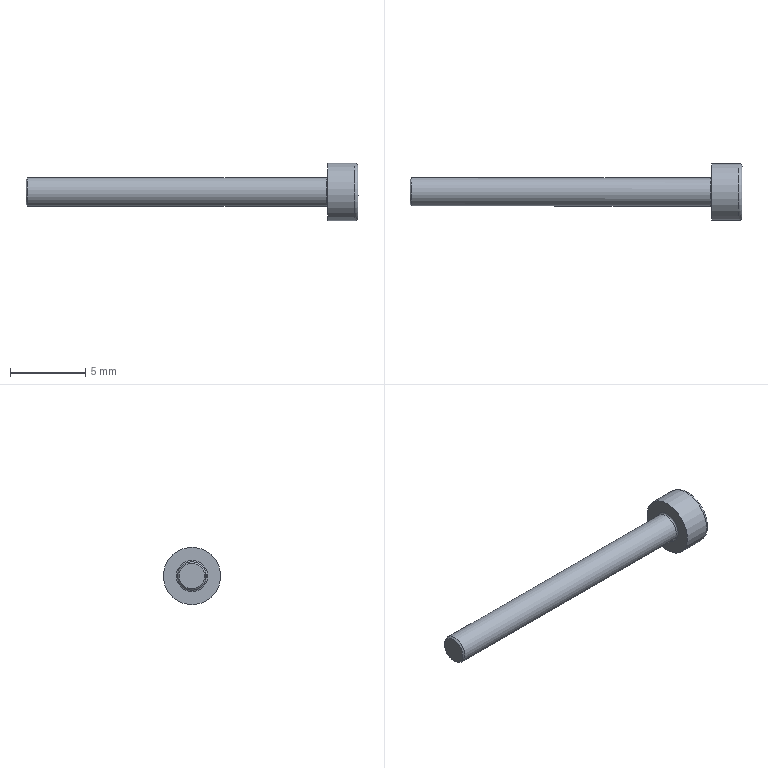Component | NX | GB-T70_1-2000_M2X20 | 1 solid | 27 faces | volume 75 mm3 | plane 15 | cone 8 | cylinder 2 | torus 2 | commonest cylinder face diameters 1.886 x1 3.8 x1